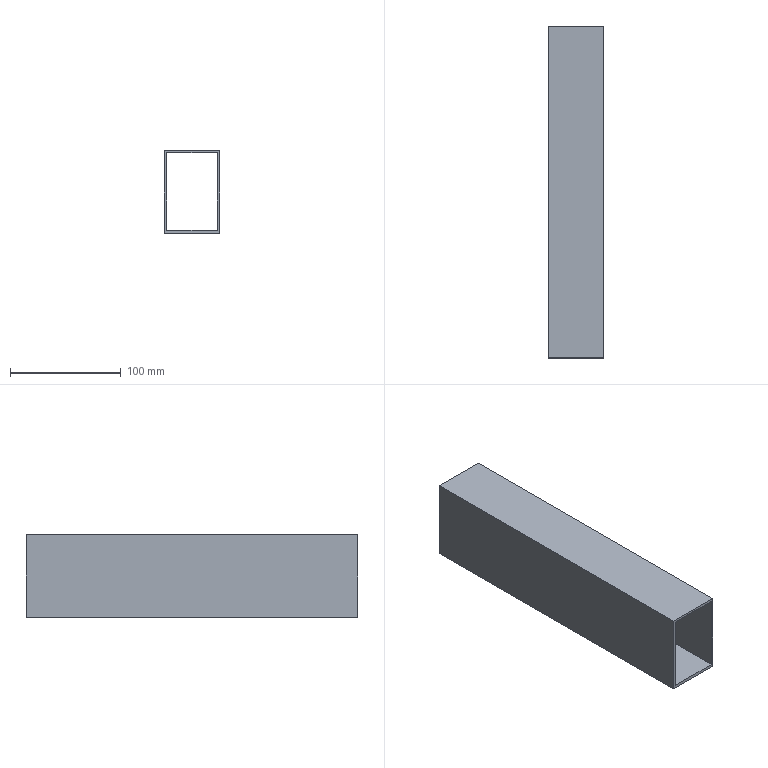Component | SolidWorks | Telescopic1-1 | 1 solid | 10 faces | box 50 x 300 x 75 mm | volume 159000 mm3 | plane 10
build123d program:
from build123d import *

# Parameters (mm, degrees)
SKETCH1_W           = 75
SKETCH1_H           = 50
BOSS_EXTRUDE1_DEPTH = 300
SKETCH2_W           = 70
SKETCH2_H           = 46
CUT_EXTRUDE1_DEPTH  = 500


with BuildPart() as part:
    # Sketch1 → Boss-Extrude1 (new body)
    with BuildSketch(Plane.XY):
        Rectangle(SKETCH1_W, SKETCH1_H)
    extrude(amount=BOSS_EXTRUDE1_DEPTH)

    # Sketch2 → Cut-Extrude1 (cut)
    with BuildSketch(Plane(origin=(0, 0, 0), x_dir=(-1, 0, 0), z_dir=(0, 0, -1))):
        with Locations((0.5, 0)):
            Rectangle(SKETCH2_W, SKETCH2_H)
    extrude(amount=-CUT_EXTRUDE1_DEPTH, mode=Mode.SUBTRACT)


solid = part.part

# Placed as in the assembly
solid = solid.moved(Location((-234.371, -636.122, 101.81), (90, 0, -90)))
STEP:
#1=CARTESIAN_POINT('',(-8.243,-36.855,2.532));
#2=VERTEX_POINT('',#1);
#3=CARTESIAN_POINT('',(-10.211,-36.855,2.532));
#4=VERTEX_POINT('',#3);
#5=CARTESIAN_POINT('',(-8.243,-36.855,2.532));
#6=DIRECTION('',(-1.,-0.,-0.));
#7=VECTOR('',#6,39.37);
#8=LINE('',#5,#7);
#9=EDGE_CURVE('',#2,#4,#8,.T.);
#10=ORIENTED_EDGE('',*,*,#9,.T.);
#11=CARTESIAN_POINT('',(-10.211,-25.044,2.532));
#12=VERTEX_POINT('',#11);
#13=CARTESIAN_POINT('',(-10.211,-25.044,2.532));
#14=DIRECTION('',(0.,-1.,0.));
#15=VECTOR('',#14,39.37);
#16=LINE('',#13,#15);
#17=EDGE_CURVE('',#12,#4,#16,.T.);
#18=ORIENTED_EDGE('',*,*,#17,.F.);
#19=CARTESIAN_POINT('',(-8.243,-25.044,2.532));
#20=VERTEX_POINT('',#19);
#21=CARTESIAN_POINT('',(-8.243,-25.044,2.532));
#22=DIRECTION('',(-1.,-0.,-0.));
#23=VECTOR('',#22,39.37);
#24=LINE('',#21,#23);
#25=EDGE_CURVE('',#20,#12,#24,.T.);
#26=ORIENTED_EDGE('',*,*,#25,.F.);
#27=CARTESIAN_POINT('',(-8.243,-25.044,2.532));
#28=DIRECTION('',(0.,-1.,0.));
#29=VECTOR('',#28,39.37);
#30=LINE('',#27,#29);
#31=EDGE_CURVE('',#20,#2,#30,.T.);
#32=ORIENTED_EDGE('',*,*,#31,.T.);
#33=EDGE_LOOP('',(#10,#18,#26,#32));
#34=FACE_OUTER_BOUND('',#33,.T.);
#35=CARTESIAN_POINT('',(-8.243,-25.044,2.532));
#36=DIRECTION('',(0.,0.,1.));
#37=DIRECTION('',(-0.,1.,-0.));
#38=AXIS2_PLACEMENT_3D('',#35,#36,#37);
#39=PLANE('',#38);
#40=ADVANCED_FACE('',(#34),#39,.F.);
#41=CARTESIAN_POINT('',(-10.211,-36.855,5.485));
#42=VERTEX_POINT('',#41);
#43=CARTESIAN_POINT('',(-10.211,-36.855,5.485));
#44=DIRECTION('',(0.,0.,1.));
#45=VECTOR('',#44,39.37);
#46=LINE('',#43,#45);
#47=EDGE_CURVE('',#4,#42,#46,.T.);
#48=ORIENTED_EDGE('',*,*,#47,.T.);
#49=CARTESIAN_POINT('',(-10.211,-25.044,5.485));
#50=VERTEX_POINT('',#49);
#51=CARTESIAN_POINT('',(-10.211,-25.044,5.485));
#52=DIRECTION('',(0.,-1.,0.));
#53=VECTOR('',#52,39.37);
#54=LINE('',#51,#53);
#55=EDGE_CURVE('',#50,#42,#54,.T.);
#56=ORIENTED_EDGE('',*,*,#55,.F.);
#57=CARTESIAN_POINT('',(-10.211,-25.044,5.485));
#58=DIRECTION('',(0.,0.,1.));
#59=VECTOR('',#58,39.37);
#60=LINE('',#57,#59);
#61=EDGE_CURVE('',#12,#50,#60,.T.);
#62=ORIENTED_EDGE('',*,*,#61,.F.);
#63=ORIENTED_EDGE('',*,*,#17,.T.);
#64=EDGE_LOOP('',(#48,#56,#62,#63));
#65=FACE_OUTER_BOUND('',#64,.T.);
#66=CARTESIAN_POINT('',(-10.211,-25.044,5.485));
#67=DIRECTION('',(1.,0.,0.));
#68=DIRECTION('',(0.,-1.,0.));
#69=AXIS2_PLACEMENT_3D('',#66,#67,#68);
#70=PLANE('',#69);
#71=ADVANCED_FACE('',(#65),#70,.F.);
#72=CARTESIAN_POINT('',(-8.243,-36.855,5.485));
#73=VERTEX_POINT('',#72);
#74=CARTESIAN_POINT('',(-8.243,-36.855,5.485));
#75=DIRECTION('',(1.,0.,0.));
#76=VECTOR('',#75,39.37);
#77=LINE('',#74,#76);
#78=EDGE_CURVE('',#42,#73,#77,.T.);
#79=ORIENTED_EDGE('',*,*,#78,.T.);
#80=CARTESIAN_POINT('',(-8.243,-25.044,5.485));
#81=VERTEX_POINT('',#80);
#82=CARTESIAN_POINT('',(-8.243,-25.044,5.485));
#83=DIRECTION('',(0.,-1.,0.));
#84=VECTOR('',#83,39.37);
#85=LINE('',#82,#84);
#86=EDGE_CURVE('',#81,#73,#85,.T.);
#87=ORIENTED_EDGE('',*,*,#86,.F.);
#88=CARTESIAN_POINT('',(-8.243,-25.044,5.485));
#89=DIRECTION('',(1.,0.,0.));
#90=VECTOR('',#89,39.37);
#91=LINE('',#88,#90);
#92=EDGE_CURVE('',#50,#81,#91,.T.);
#93=ORIENTED_EDGE('',*,*,#92,.F.);
#94=ORIENTED_EDGE('',*,*,#55,.T.);
#95=EDGE_LOOP('',(#79,#87,#93,#94));
#96=FACE_OUTER_BOUND('',#95,.T.);
#97=CARTESIAN_POINT('',(-8.243,-25.044,5.485));
#98=DIRECTION('',(-0.,-0.,-1.));
#99=DIRECTION('',(0.,-1.,0.));
#100=AXIS2_PLACEMENT_3D('',#97,#98,#99);
#101=PLANE('',#100);
#102=ADVANCED_FACE('',(#96),#101,.F.);
#103=CARTESIAN_POINT('',(-8.243,-36.855,5.485));
#104=DIRECTION('',(-0.,-0.,-1.));
#105=VECTOR('',#104,39.37);
#106=LINE('',#103,#105);
#107=EDGE_CURVE('',#73,#2,#106,.T.);
#108=ORIENTED_EDGE('',*,*,#107,.T.);
#109=ORIENTED_EDGE('',*,*,#31,.F.);
#110=CARTESIAN_POINT('',(-8.243,-25.044,5.485));
#111=DIRECTION('',(-0.,-0.,-1.));
#112=VECTOR('',#111,39.37);
#113=LINE('',#110,#112);
#114=EDGE_CURVE('',#81,#20,#113,.T.);
#115=ORIENTED_EDGE('',*,*,#114,.F.);
#116=ORIENTED_EDGE('',*,*,#86,.T.);
#117=EDGE_LOOP('',(#108,#109,#115,#116));
#118=FACE_OUTER_BOUND('',#117,.T.);
#119=CARTESIAN_POINT('',(-8.243,-25.044,5.485));
#120=DIRECTION('',(-1.,-0.,-0.));
#121=DIRECTION('',(-0.,1.,-0.));
#122=AXIS2_PLACEMENT_3D('',#119,#120,#121);
#123=PLANE('',#122);
#124=ADVANCED_FACE('',(#118),#123,.F.);
#125=CARTESIAN_POINT('',(-10.133,-25.044,5.406));
#126=VERTEX_POINT('',#125);
#127=CARTESIAN_POINT('',(-10.133,-25.044,2.65));
#128=VERTEX_POINT('',#127);
#129=CARTESIAN_POINT('',(-10.133,-25.044,4.008));
#130=DIRECTION('',(-0.,-0.,-1.));
#131=VECTOR('',#130,39.37);
#132=LINE('',#129,#131);
#133=EDGE_CURVE('',#126,#128,#132,.T.);
#134=ORIENTED_EDGE('',*,*,#133,.T.);
#135=CARTESIAN_POINT('',(-8.322,-25.044,2.65));
#136=VERTEX_POINT('',#135);
#137=CARTESIAN_POINT('',(-9.227,-25.044,2.65));
#138=DIRECTION('',(1.,0.,0.));
#139=VECTOR('',#138,39.37);
#140=LINE('',#137,#139);
#141=EDGE_CURVE('',#128,#136,#140,.T.);
#142=ORIENTED_EDGE('',*,*,#141,.T.);
#143=CARTESIAN_POINT('',(-8.322,-25.044,5.406));
#144=VERTEX_POINT('',#143);
#145=CARTESIAN_POINT('',(-8.322,-25.044,4.008));
#146=DIRECTION('',(0.,0.,1.));
#147=VECTOR('',#146,39.37);
#148=LINE('',#145,#147);
#149=EDGE_CURVE('',#136,#144,#148,.T.);
#150=ORIENTED_EDGE('',*,*,#149,.T.);
#151=CARTESIAN_POINT('',(-9.227,-25.044,5.406));
#152=DIRECTION('',(-1.,-0.,-0.));
#153=VECTOR('',#152,39.37);
#154=LINE('',#151,#153);
#155=EDGE_CURVE('',#144,#126,#154,.T.);
#156=ORIENTED_EDGE('',*,*,#155,.T.);
#157=EDGE_LOOP('',(#134,#142,#150,#156));
#158=FACE_BOUND('',#157,.T.);
#159=ORIENTED_EDGE('',*,*,#25,.T.);
#160=ORIENTED_EDGE('',*,*,#61,.T.);
#161=ORIENTED_EDGE('',*,*,#92,.T.);
#162=ORIENTED_EDGE('',*,*,#114,.T.);
#163=EDGE_LOOP('',(#159,#160,#161,#162));
#164=FACE_OUTER_BOUND('',#163,.T.);
#165=CARTESIAN_POINT('',(-9.227,-25.044,4.008));
#166=DIRECTION('',(0.,-1.,0.));
#167=DIRECTION('',(0.,0.,1.));
#168=AXIS2_PLACEMENT_3D('',#165,#166,#167);
#169=PLANE('',#168);
#170=ADVANCED_FACE('',(#158,#164),#169,.F.);
#171=CARTESIAN_POINT('',(-10.133,-36.855,2.65));
#172=VERTEX_POINT('',#171);
#173=CARTESIAN_POINT('',(-8.322,-36.855,2.65));
#174=VERTEX_POINT('',#173);
#175=CARTESIAN_POINT('',(-10.133,-36.855,2.65));
#176=DIRECTION('',(1.,0.,0.));
#177=VECTOR('',#176,39.37);
#178=LINE('',#175,#177);
#179=EDGE_CURVE('',#172,#174,#178,.T.);
#180=ORIENTED_EDGE('',*,*,#179,.F.);
#181=CARTESIAN_POINT('',(-10.133,-36.855,5.406));
#182=VERTEX_POINT('',#181);
#183=CARTESIAN_POINT('',(-10.133,-36.855,2.65));
#184=DIRECTION('',(-0.,-0.,-1.));
#185=VECTOR('',#184,39.37);
#186=LINE('',#183,#185);
#187=EDGE_CURVE('',#182,#172,#186,.T.);
#188=ORIENTED_EDGE('',*,*,#187,.F.);
#189=CARTESIAN_POINT('',(-8.322,-36.855,5.406));
#190=VERTEX_POINT('',#189);
#191=CARTESIAN_POINT('',(-10.133,-36.855,5.406));
#192=DIRECTION('',(-1.,-0.,-0.));
#193=VECTOR('',#192,39.37);
#194=LINE('',#191,#193);
#195=EDGE_CURVE('',#190,#182,#194,.T.);
#196=ORIENTED_EDGE('',*,*,#195,.F.);
#197=CARTESIAN_POINT('',(-8.322,-36.855,2.65));
#198=DIRECTION('',(0.,0.,1.));
#199=VECTOR('',#198,39.37);
#200=LINE('',#197,#199);
#201=EDGE_CURVE('',#174,#190,#200,.T.);
#202=ORIENTED_EDGE('',*,*,#201,.F.);
#203=EDGE_LOOP('',(#180,#188,#196,#202));
#204=FACE_BOUND('',#203,.T.);
#205=ORIENTED_EDGE('',*,*,#9,.F.);
#206=ORIENTED_EDGE('',*,*,#107,.F.);
#207=ORIENTED_EDGE('',*,*,#78,.F.);
#208=ORIENTED_EDGE('',*,*,#47,.F.);
#209=EDGE_LOOP('',(#205,#206,#207,#208));
#210=FACE_OUTER_BOUND('',#209,.T.);
#211=CARTESIAN_POINT('',(-9.227,-36.855,4.008));
#212=DIRECTION('',(0.,-1.,0.));
#213=DIRECTION('',(0.,0.,1.));
#214=AXIS2_PLACEMENT_3D('',#211,#212,#213);
#215=PLANE('',#214);
#216=ADVANCED_FACE('',(#204,#210),#215,.T.);
#217=CARTESIAN_POINT('',(-10.133,-17.17,2.65));
#218=DIRECTION('',(0.,-1.,0.));
#219=VECTOR('',#218,39.37);
#220=LINE('',#217,#219);
#221=EDGE_CURVE('',#128,#172,#220,.T.);
#222=ORIENTED_EDGE('',*,*,#221,.T.);
#223=ORIENTED_EDGE('',*,*,#179,.T.);
#224=CARTESIAN_POINT('',(-8.322,-17.17,2.65));
#225=DIRECTION('',(0.,-1.,0.));
#226=VECTOR('',#225,39.37);
#227=LINE('',#224,#226);
#228=EDGE_CURVE('',#136,#174,#227,.T.);
#229=ORIENTED_EDGE('',*,*,#228,.F.);
#230=ORIENTED_EDGE('',*,*,#141,.F.);
#231=EDGE_LOOP('',(#222,#223,#229,#230));
#232=FACE_OUTER_BOUND('',#231,.T.);
#233=CARTESIAN_POINT('',(-10.133,-17.17,2.65));
#234=DIRECTION('',(0.,-0.,-1.));
#235=DIRECTION('',(-1.,-0.,-0.));
#236=AXIS2_PLACEMENT_3D('',#233,#234,#235);
#237=PLANE('',#236);
#238=ADVANCED_FACE('',(#232),#237,.F.);
#239=CARTESIAN_POINT('',(-10.133,-17.17,5.406));
#240=DIRECTION('',(0.,-1.,0.));
#241=VECTOR('',#240,39.37);
#242=LINE('',#239,#241);
#243=EDGE_CURVE('',#126,#182,#242,.T.);
#244=ORIENTED_EDGE('',*,*,#243,.T.);
#245=ORIENTED_EDGE('',*,*,#187,.T.);
#246=ORIENTED_EDGE('',*,*,#221,.F.);
#247=ORIENTED_EDGE('',*,*,#133,.F.);
#248=EDGE_LOOP('',(#244,#245,#246,#247));
#249=FACE_OUTER_BOUND('',#248,.T.);
#250=CARTESIAN_POINT('',(-10.133,-17.17,2.65));
#251=DIRECTION('',(-1.,-0.,-0.));
#252=DIRECTION('',(-0.,1.,-0.));
#253=AXIS2_PLACEMENT_3D('',#250,#251,#252);
#254=PLANE('',#253);
#255=ADVANCED_FACE('',(#249),#254,.F.);
#256=CARTESIAN_POINT('',(-8.322,-17.17,5.406));
#257=DIRECTION('',(0.,-1.,0.));
#258=VECTOR('',#257,39.37);
#259=LINE('',#256,#258);
#260=EDGE_CURVE('',#144,#190,#259,.T.);
#261=ORIENTED_EDGE('',*,*,#260,.T.);
#262=ORIENTED_EDGE('',*,*,#195,.T.);
#263=ORIENTED_EDGE('',*,*,#243,.F.);
#264=ORIENTED_EDGE('',*,*,#155,.F.);
#265=EDGE_LOOP('',(#261,#262,#263,#264));
#266=FACE_OUTER_BOUND('',#265,.T.);
#267=CARTESIAN_POINT('',(-10.133,-17.17,5.406));
#268=DIRECTION('',(-0.,0.,1.));
#269=DIRECTION('',(1.,0.,0.));
#270=AXIS2_PLACEMENT_3D('',#267,#268,#269);
#271=PLANE('',#270);
#272=ADVANCED_FACE('',(#266),#271,.F.);
#273=ORIENTED_EDGE('',*,*,#228,.T.);
#274=ORIENTED_EDGE('',*,*,#201,.T.);
#275=ORIENTED_EDGE('',*,*,#260,.F.);
#276=ORIENTED_EDGE('',*,*,#149,.F.);
#277=EDGE_LOOP('',(#273,#274,#275,#276));
#278=FACE_OUTER_BOUND('',#277,.T.);
#279=CARTESIAN_POINT('',(-8.322,-17.17,2.65));
#280=DIRECTION('',(1.,0.,0.));
#281=DIRECTION('',(0.,-1.,0.));
#282=AXIS2_PLACEMENT_3D('',#279,#280,#281);
#283=PLANE('',#282);
#284=ADVANCED_FACE('',(#278),#283,.F.);
#285=CLOSED_SHELL('',(#40,#71,#102,#124,#170,#216,#238,#255,#272,#284));
#286=MANIFOLD_SOLID_BREP('',#285);
#287=CARTESIAN_POINT('',(0.,0.,0.));
#288=DIRECTION('',(0.,0.,1.));
#289=DIRECTION('',(1.,0.,0.));
#290=AXIS2_PLACEMENT_3D('',#287,#288,#289);
#291=(LENGTH_UNIT()NAMED_UNIT(*)SI_UNIT($,.METRE.));
#292=LENGTH_MEASURE_WITH_UNIT(LENGTH_MEASURE(0.0254),#291);
#293=DIMENSIONAL_EXPONENTS(1.,0.,0.,0.,0.,0.,0.);
#294=(CONVERSION_BASED_UNIT('',#292)LENGTH_UNIT()NAMED_UNIT(#293));
#295=UNCERTAINTY_MEASURE_WITH_UNIT(LENGTH_MEASURE(0.00001),#294,'','');
#296=(NAMED_UNIT(*)PLANE_ANGLE_UNIT()SI_UNIT($,.RADIAN.));
#297=(NAMED_UNIT(*)SI_UNIT($,.STERADIAN.)SOLID_ANGLE_UNIT());
#298=(GEOMETRIC_REPRESENTATION_CONTEXT(3)GLOBAL_UNCERTAINTY_ASSIGNED_CONTEXT((#295))GLOBAL_UNIT_ASSIGNED_CONTEXT((#294,#296,#297))REPRESENTATION_CONTEXT('',''));
#299=ADVANCED_BREP_SHAPE_REPRESENTATION('',(#286,#290),#298);
#300=COLOUR_RGB('',0.7922,0.8196,0.9333);
#301=FILL_AREA_STYLE_COLOUR('',#300);
#302=FILL_AREA_STYLE('',(#301));
#303=SURFACE_STYLE_FILL_AREA(#302);
#304=SURFACE_SIDE_STYLE('',(#303));
#305=SURFACE_STYLE_USAGE(.BOTH.,#304);
#306=PRESENTATION_STYLE_ASSIGNMENT((#305));
#307=STYLED_ITEM('',(#306),#286);
#308=(LENGTH_UNIT()NAMED_UNIT(*)SI_UNIT($,.METRE.));
#309=LENGTH_MEASURE_WITH_UNIT(LENGTH_MEASURE(0.0254),#308);
#310=DIMENSIONAL_EXPONENTS(1.,0.,0.,0.,0.,0.,0.);
#311=(CONVERSION_BASED_UNIT('',#309)LENGTH_UNIT()NAMED_UNIT(#310));
#312=UNCERTAINTY_MEASURE_WITH_UNIT(LENGTH_MEASURE(0.00001),#311,'','');
#313=(NAMED_UNIT(*)PLANE_ANGLE_UNIT()SI_UNIT($,.RADIAN.));
#314=(NAMED_UNIT(*)SI_UNIT($,.STERADIAN.)SOLID_ANGLE_UNIT());
#315=(GEOMETRIC_REPRESENTATION_CONTEXT(3)GLOBAL_UNCERTAINTY_ASSIGNED_CONTEXT((#312))GLOBAL_UNIT_ASSIGNED_CONTEXT((#311,#313,#314))REPRESENTATION_CONTEXT('',''));
#316=MECHANICAL_DESIGN_GEOMETRIC_PRESENTATION_REPRESENTATION('',(#307),#315);
#317=PRESENTATION_LAYER_ASSIGNMENT('','',(#307));